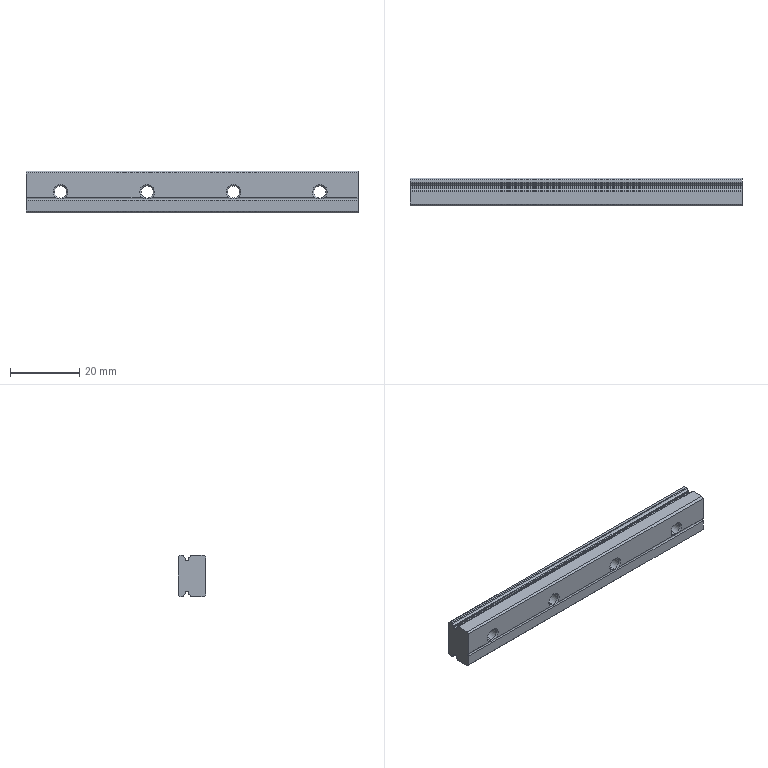Component | SolidWorks | 17268Rail-MGN12R01114HM-10_0-1 | 1 solid | 72 faces | volume 8093 mm3 | cylinder 33 | plane 23 | cone 16 | commonest cylinder face diameters 0.5 x12 3.5 x8 6 x8 2.4 x4 1 x1 | material SKD-11 HRC58° Hard Chrome Plated